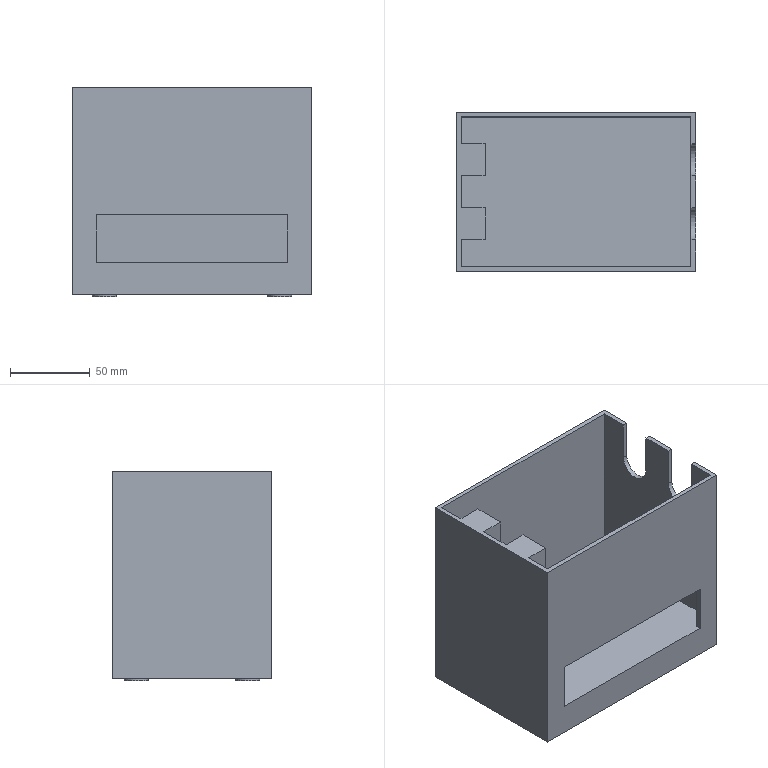Component | NX | SHE_JI-1 | 1 solid | 49 faces | volume 466077 mm3 | plane 35 | cylinder 14 | commonest cylinder face diameters 20 x4 15 x4 8 x4 12 x2